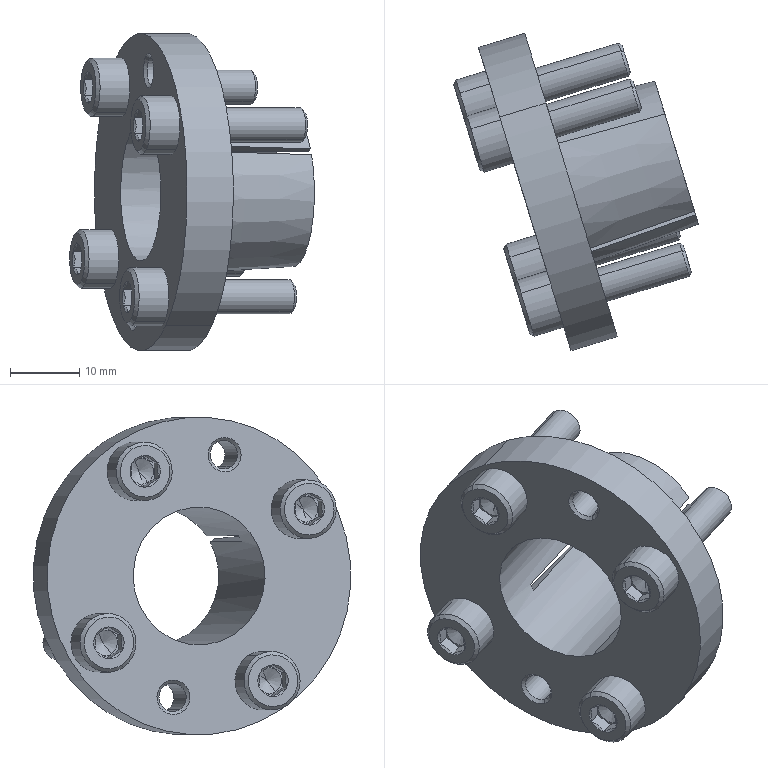Component | SolidWorks | v1ZHXTPTLA36P5M100_E_20SB1-1_v1ZHXT20SB1-1 | 1 solid | 131 faces | box 35.47 x 46.04 x 46 mm | volume 12576 mm3 | cone 63 | plane 44 | cylinder 24 | commonest cylinder face diameters 8.5 x8 5 x8 4.134 x4 46 x2 20 x2